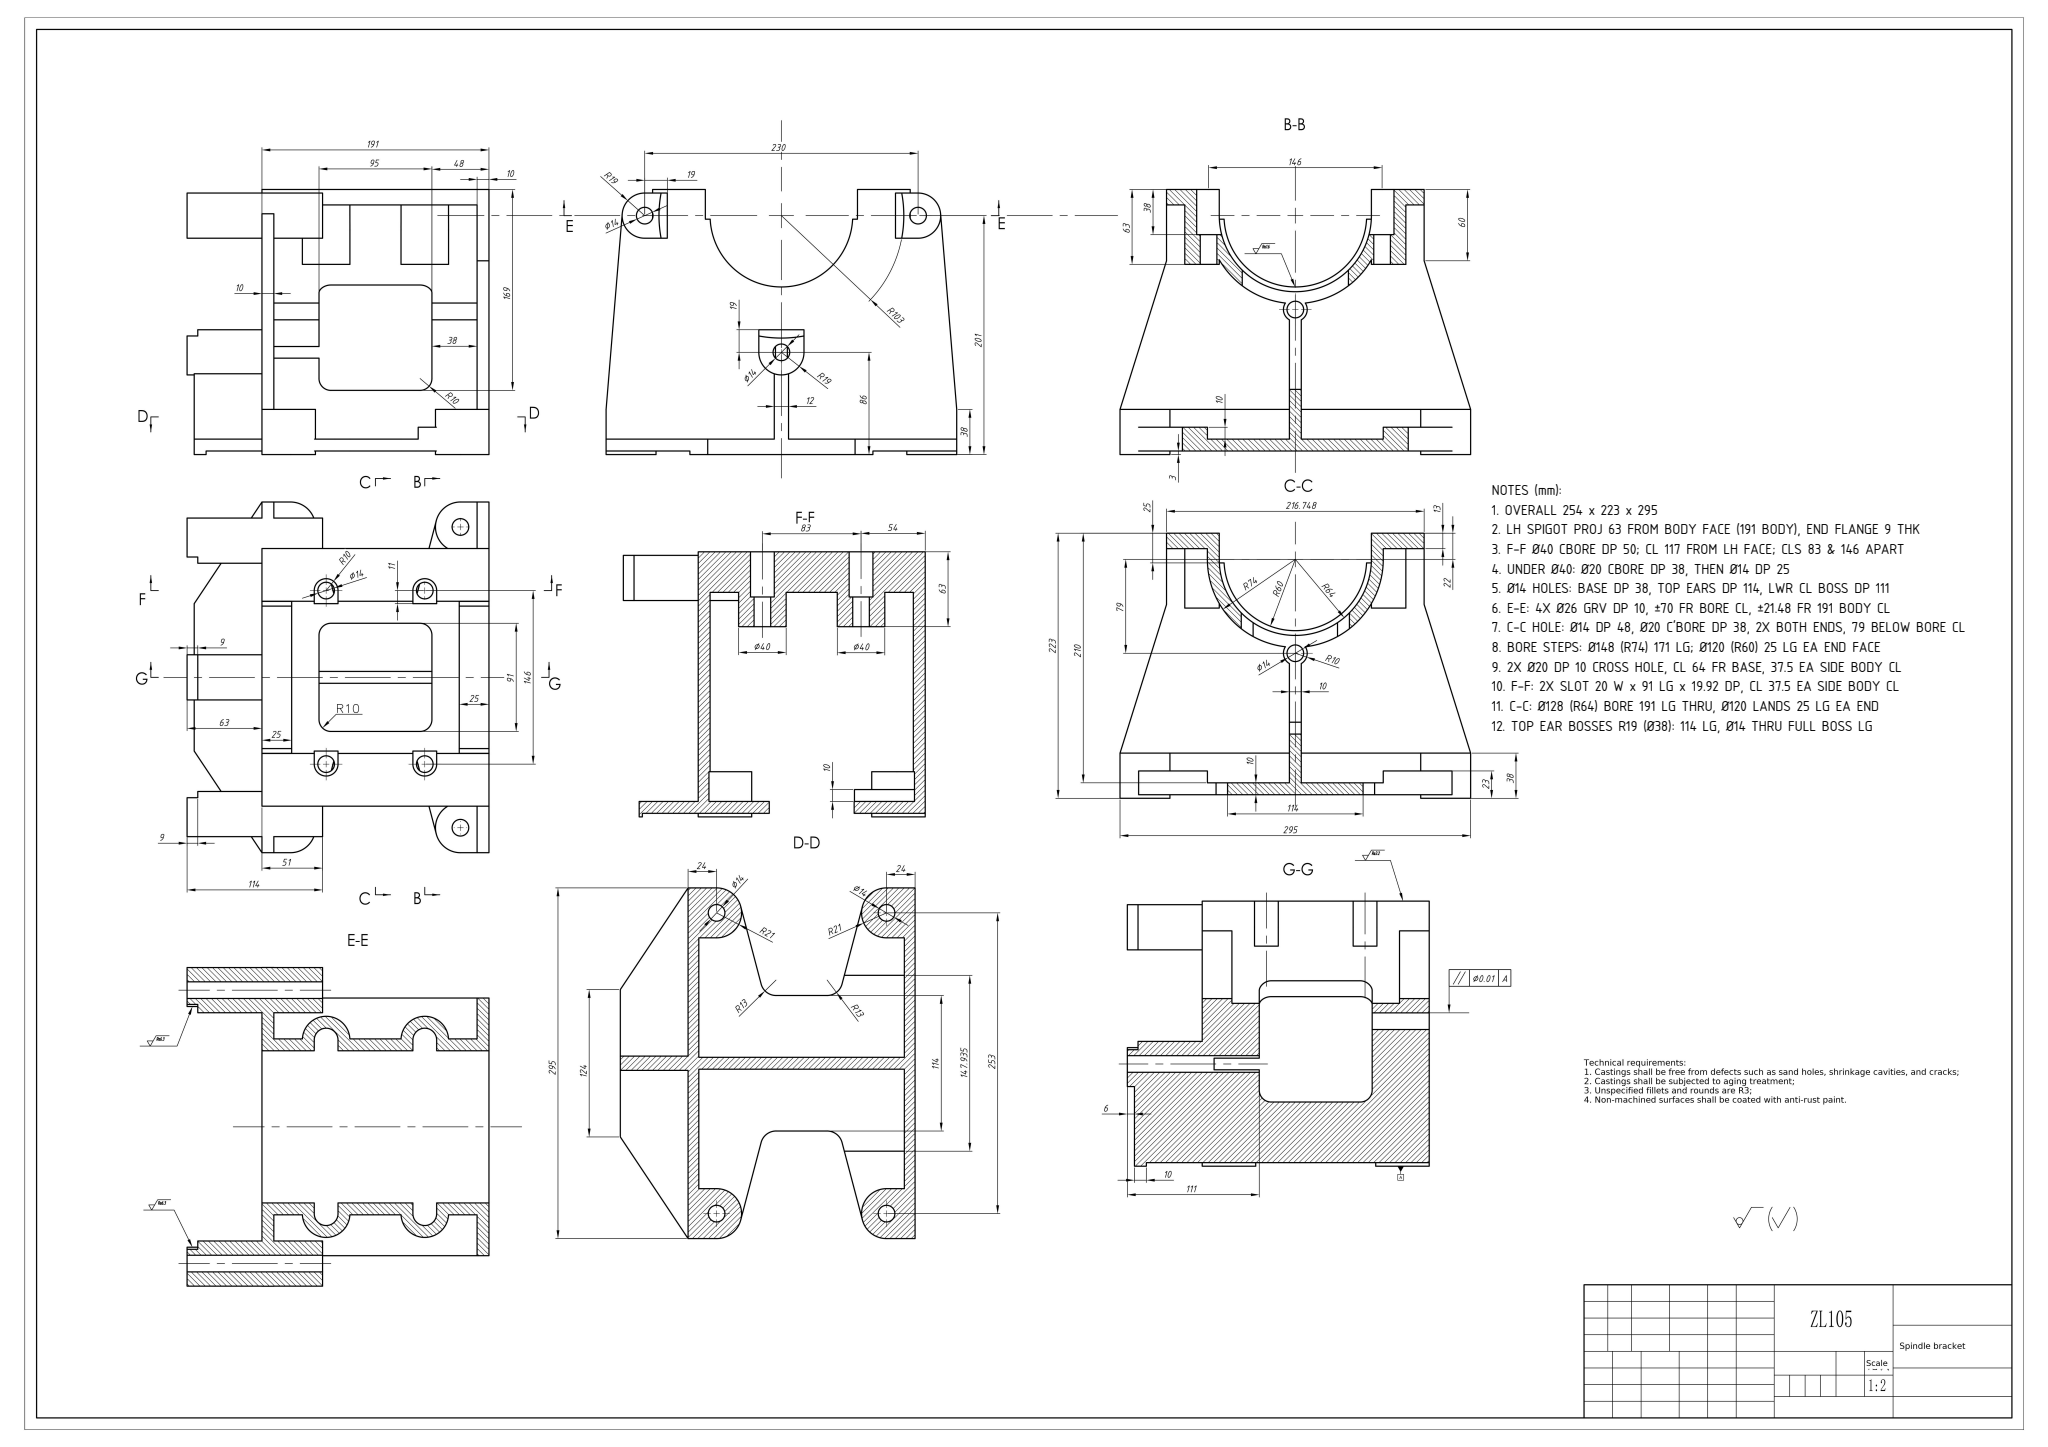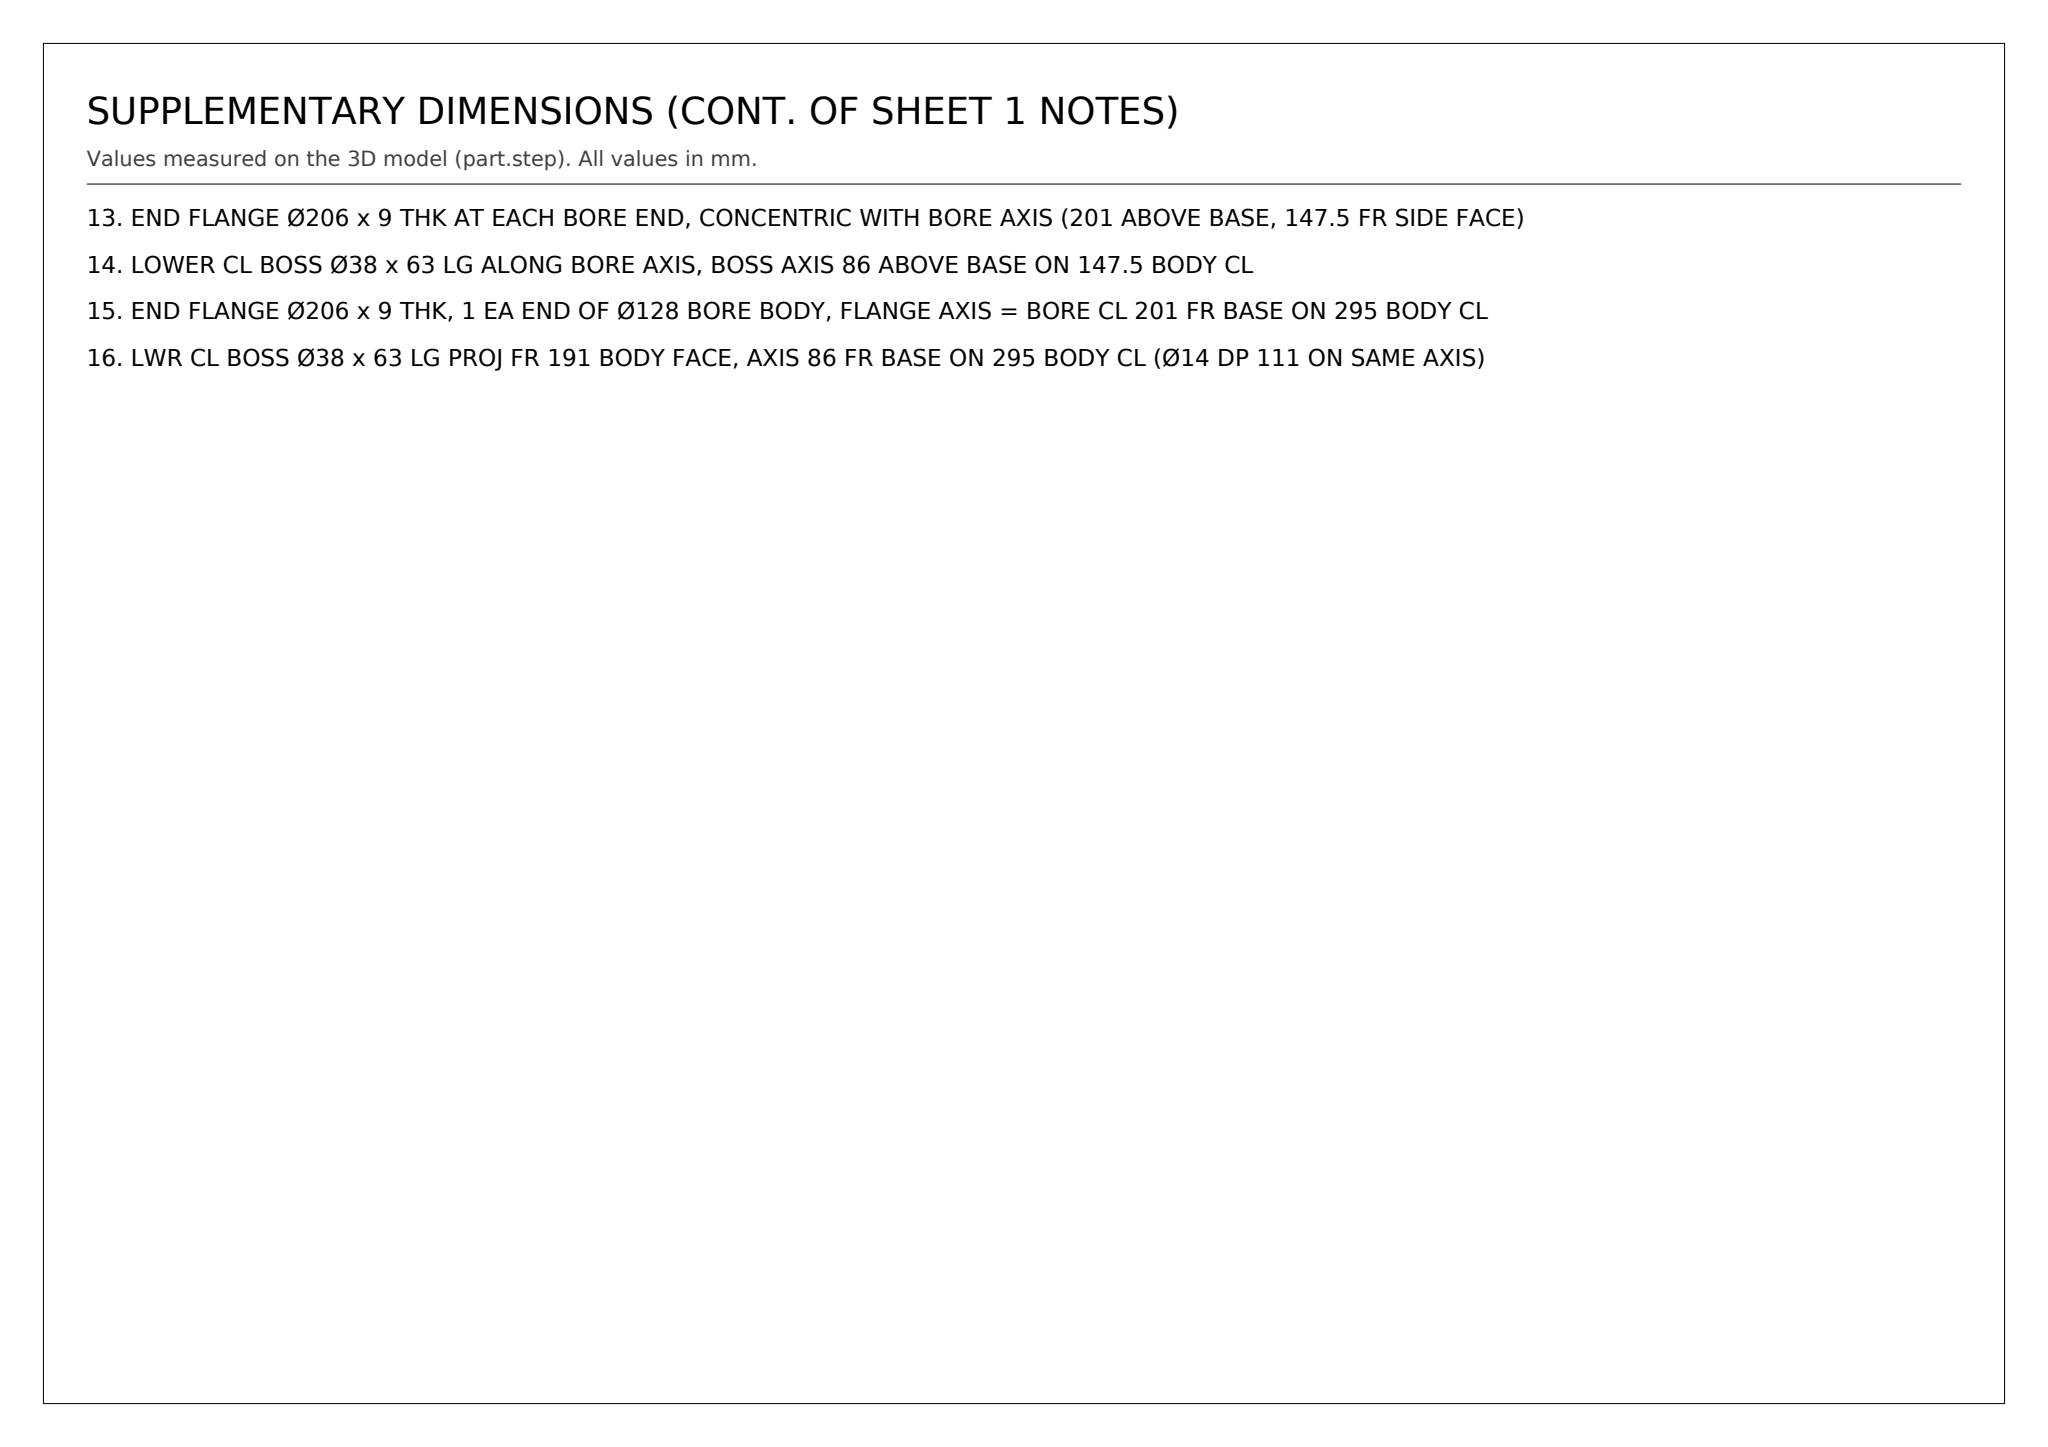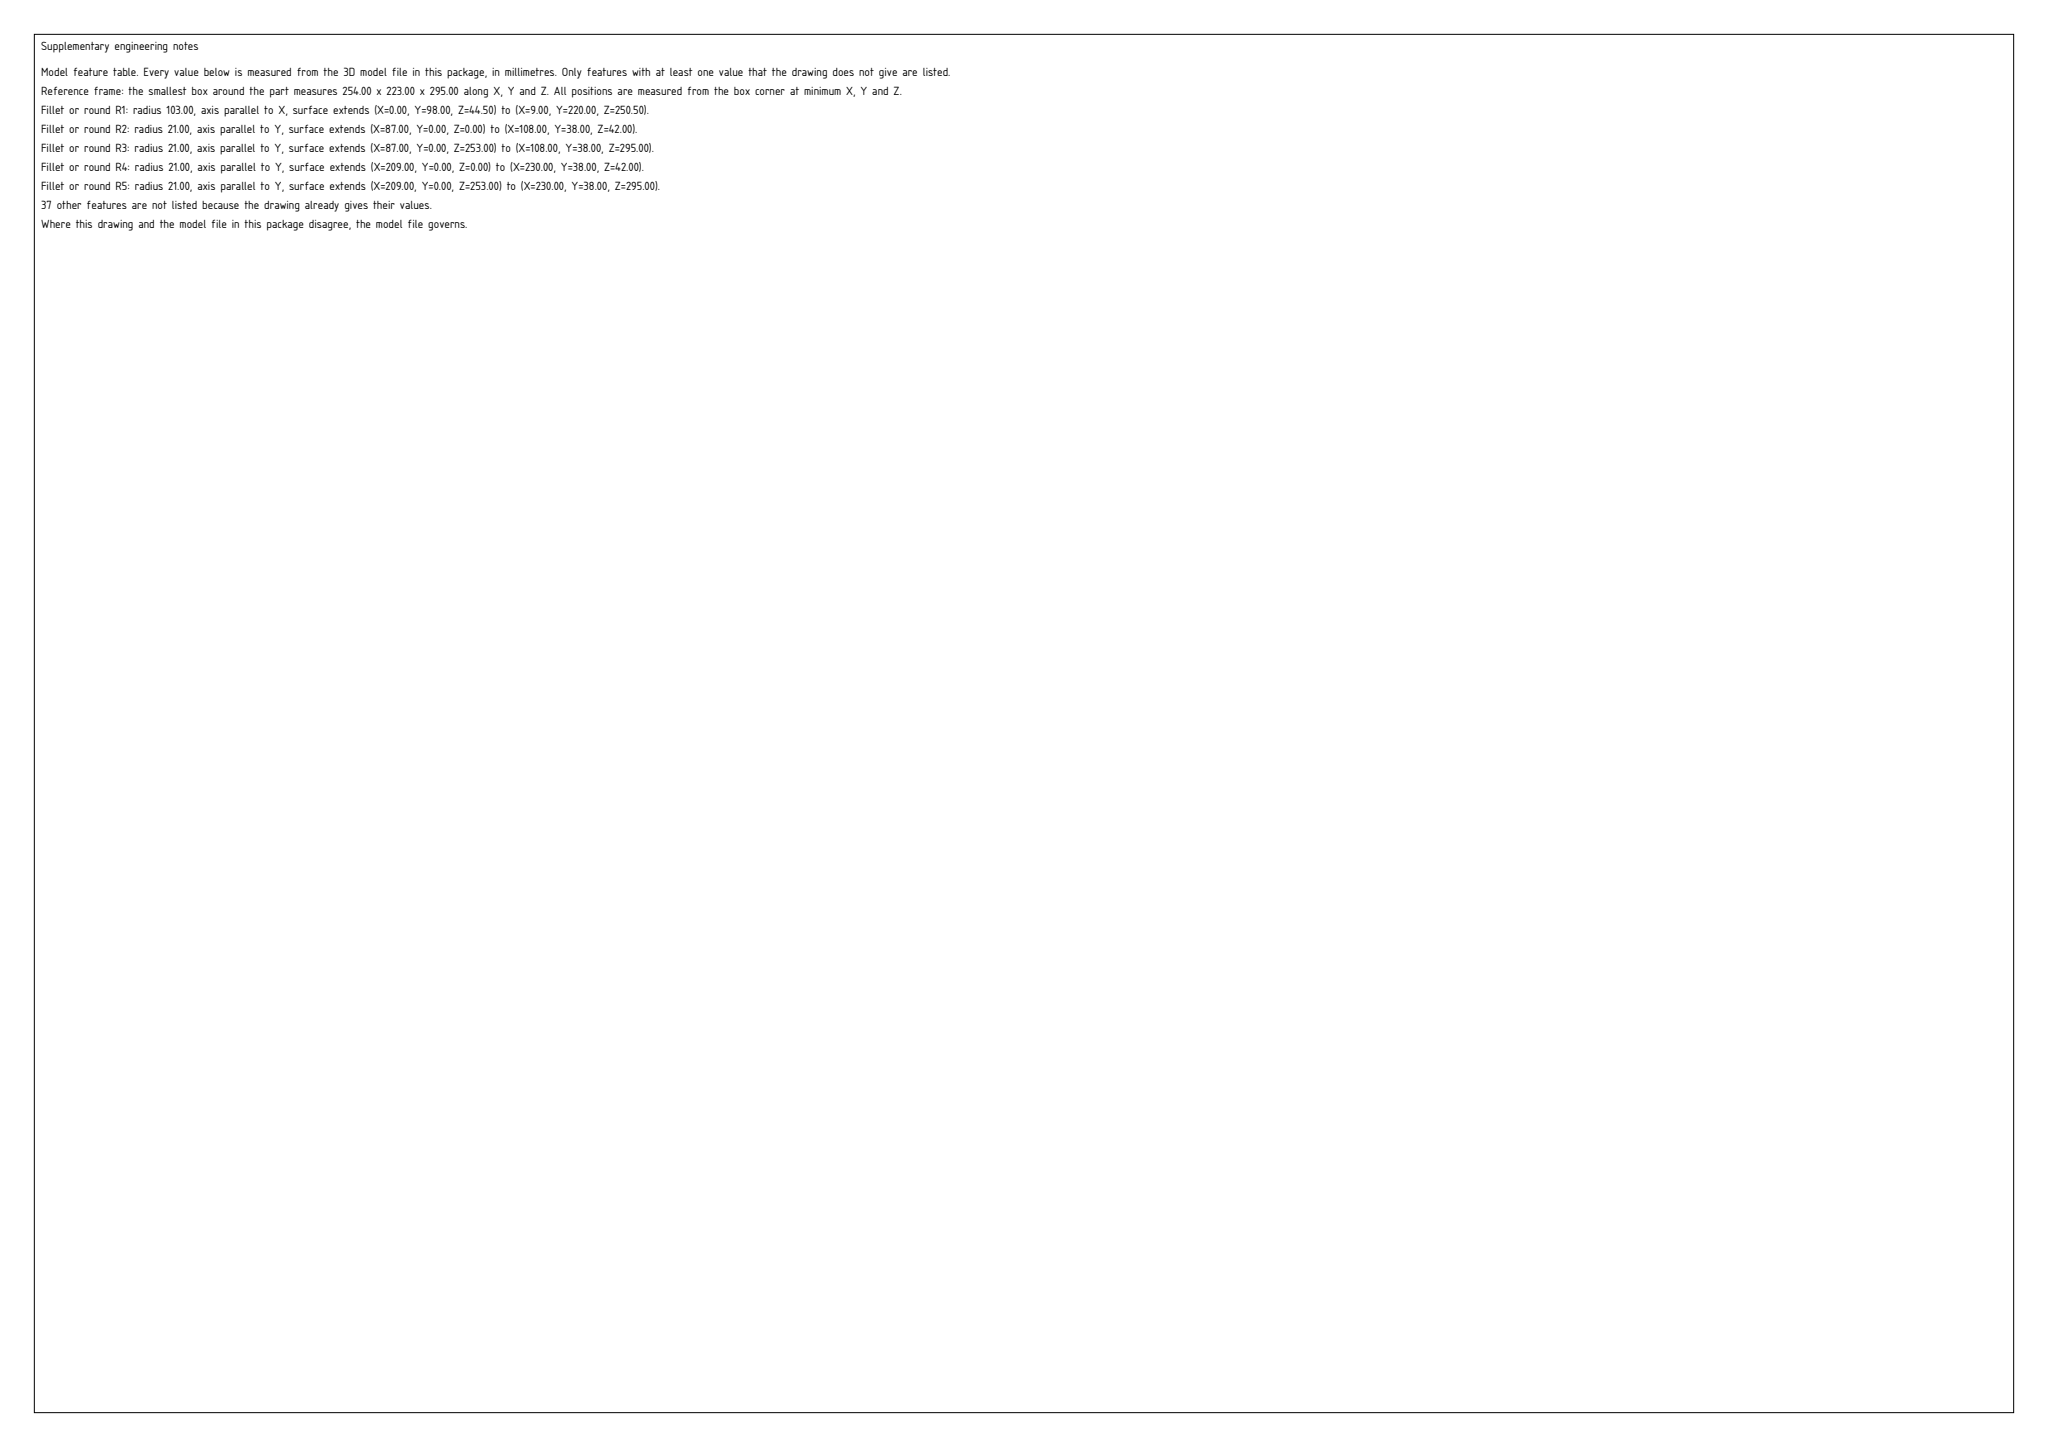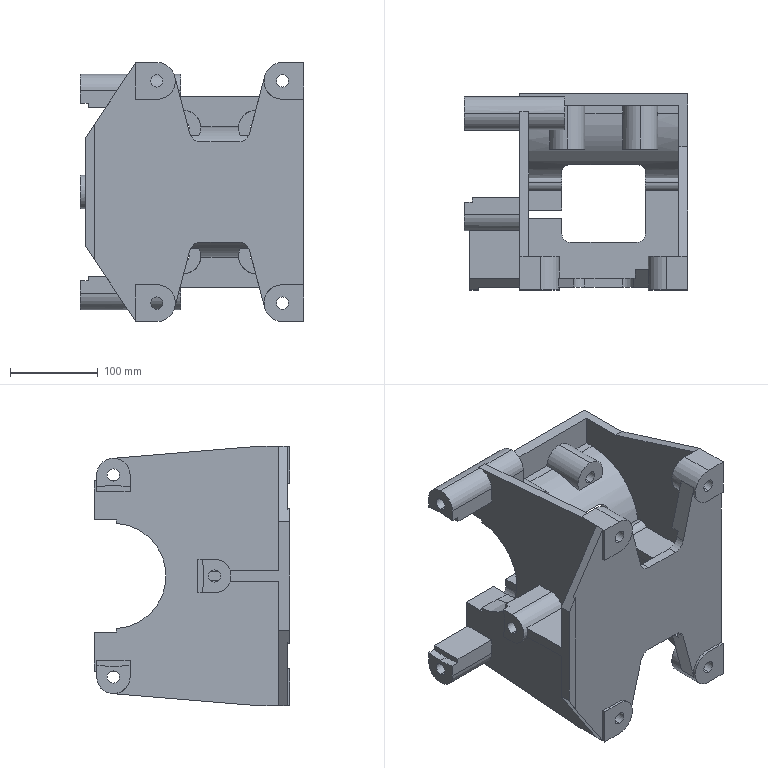Part | SolidWorks | mm | 1 solid | 211 faces | box 254 x 223 x 295 mm | volume 2667712 mm3 | plane 141 | cylinder 70 | commonest cylinder face diameters 14 x24 20 x18 40 x6 38 x5 206 x4 42 x4 26 x4 148 x2
Drawing notes:
OVERALL 254 x 223 x 295 | from the solid: bbox_xyz [254.0, 223.0, 295.0]
LH SPIGOT PROJ 63 FROM BODY FACE (191 BODY), END FLANGE 9 THK | from the solid: x planes 0, 9, 63 each count 3; 254-191=63
F-F Ø40 CBORE DP 50; CL 117 FROM LH FACE; CLS 83 & 146 APART | from the solid: Ø40 y-axis @ x=117 & 200 (83 apart), z=74.5 & 220.5 (146 apart), L=50; 254-200=54
UNDER Ø40: Ø20 CBORE DP 38, THEN Ø14 DP 25 | from the solid: Ø20 y-axis @ (117/200, 74.5/220.5) L=38; Ø14 y-axis same CLs L=25
Ø14 HOLES: BASE DP 38, TOP EARS DP 114, LWR CL BOSS DP 111 | from the solid: Ø14 y-axis @ (87/230, 21/274) L=38; Ø14 x-axis @ y201, z32.5/262.5 L=114; Ø14 x-axis @ y86, z147.5 L=111
E-E: 4X Ø26 GRV DP 10, ±70 FR BORE CL, ±21.48 FR 191 BODY CL | from the solid: cyl Ø26 axis y L=10 at x=137.02/179.98, z=77.5/217.5; bore CL z=147.5; 191 body x=63..254, mid 158.5
C-C HOLE: Ø14 DP 48, Ø20 C'BORE DP 38, 2X BOTH ENDS, 79 BELOW BORE CL | from the solid: cyl Ø14 axis x L=48 and Ø20 axis x L=38 at y=122, z=147.5; bore axis y=201 (201-122=79)
BORE STEPS: Ø148 (R74) 171 LG; Ø120 (R60) 25 LG EA END FACE | from the solid: cyl Ø148 axis x L=171 (x=73..244); cyl Ø120 axis x L=25 x2 (x=63..88 and 229..254)
2X Ø20 DP 10 CROSS HOLE, CL 64 FR BASE, 37.5 EA SIDE BODY CL | from the solid: cyl Ø20 axis z L=10 at x=121 & 196, y=64; base y=0; 191 body mid x=158.5
F-F: 2X SLOT 20 W x 91 LG x 19.92 DP, CL 37.5 EA SIDE BODY CL | from the solid: cyl Ø20 axis y L=19.92 at x=121/196, z=112 & 183 (183-112+20=91); body mid x=158.5
C-C: Ø128 (R64) BORE 191 LG THRU, Ø120 LANDS 25 LG EA END | from the solid: Cyl dia128 axis x at y201,z147.5 len191 (x=63..254, i.e. full bore-face to bore-face); dia120 axis x same axis len25 x2 at 63-88 and 229-254; dia148 outer 171 LG spans x=73..244 (x planes 63,73,88,229,244,254)
TOP EAR BOSSES R19 (Ø38): 114 LG, Ø14 THRU FULL BOSS LG | from the solid: Cyl dia38 axis x at y201,z32.5 len114 and y201,z262.5 len114; coaxial dia14 axis x len114 at both locations
END FLANGE Ø206 x 9 THK AT EACH BORE END, CONCENTRIC WITH BORE AXIS (201 ABOVE BASE, 147.5 FR SIDE FACE) | from the solid: cylinders: [206.0,"x",[null,201.0,147.5],9.0,4] (Ø206 x 9 long, bore axis)
LOWER CL BOSS Ø38 x 63 LG ALONG BORE AXIS, BOSS AXIS 86 ABOVE BASE ON 147.5 BODY CL | from the solid: cylinders: [38.0,"x",[null,86.0,147.5],63.0,1] with coaxial [14.0,"x",[null,86.0,147.5],111.0]
END FLANGE Ø206 x 9 THK, 1 EA END OF Ø128 BORE BODY, FLANGE AXIS = BORE CL 201 FR BASE ON 295 BODY CL | from the solid: cylinders[206,"x",[null,201.0,147.5],9.0] (4 faces, both bore ends)
LWR CL BOSS Ø38 x 63 LG PROJ FR 191 BODY FACE, AXIS 86 FR BASE ON 295 BODY CL (Ø14 DP 111 ON SAME AXIS) | from the solid: cylinders[38,"x",[null,86.0,147.5],63.0] with cylinders[14,"x",[null,86.0,147.5],111.0]